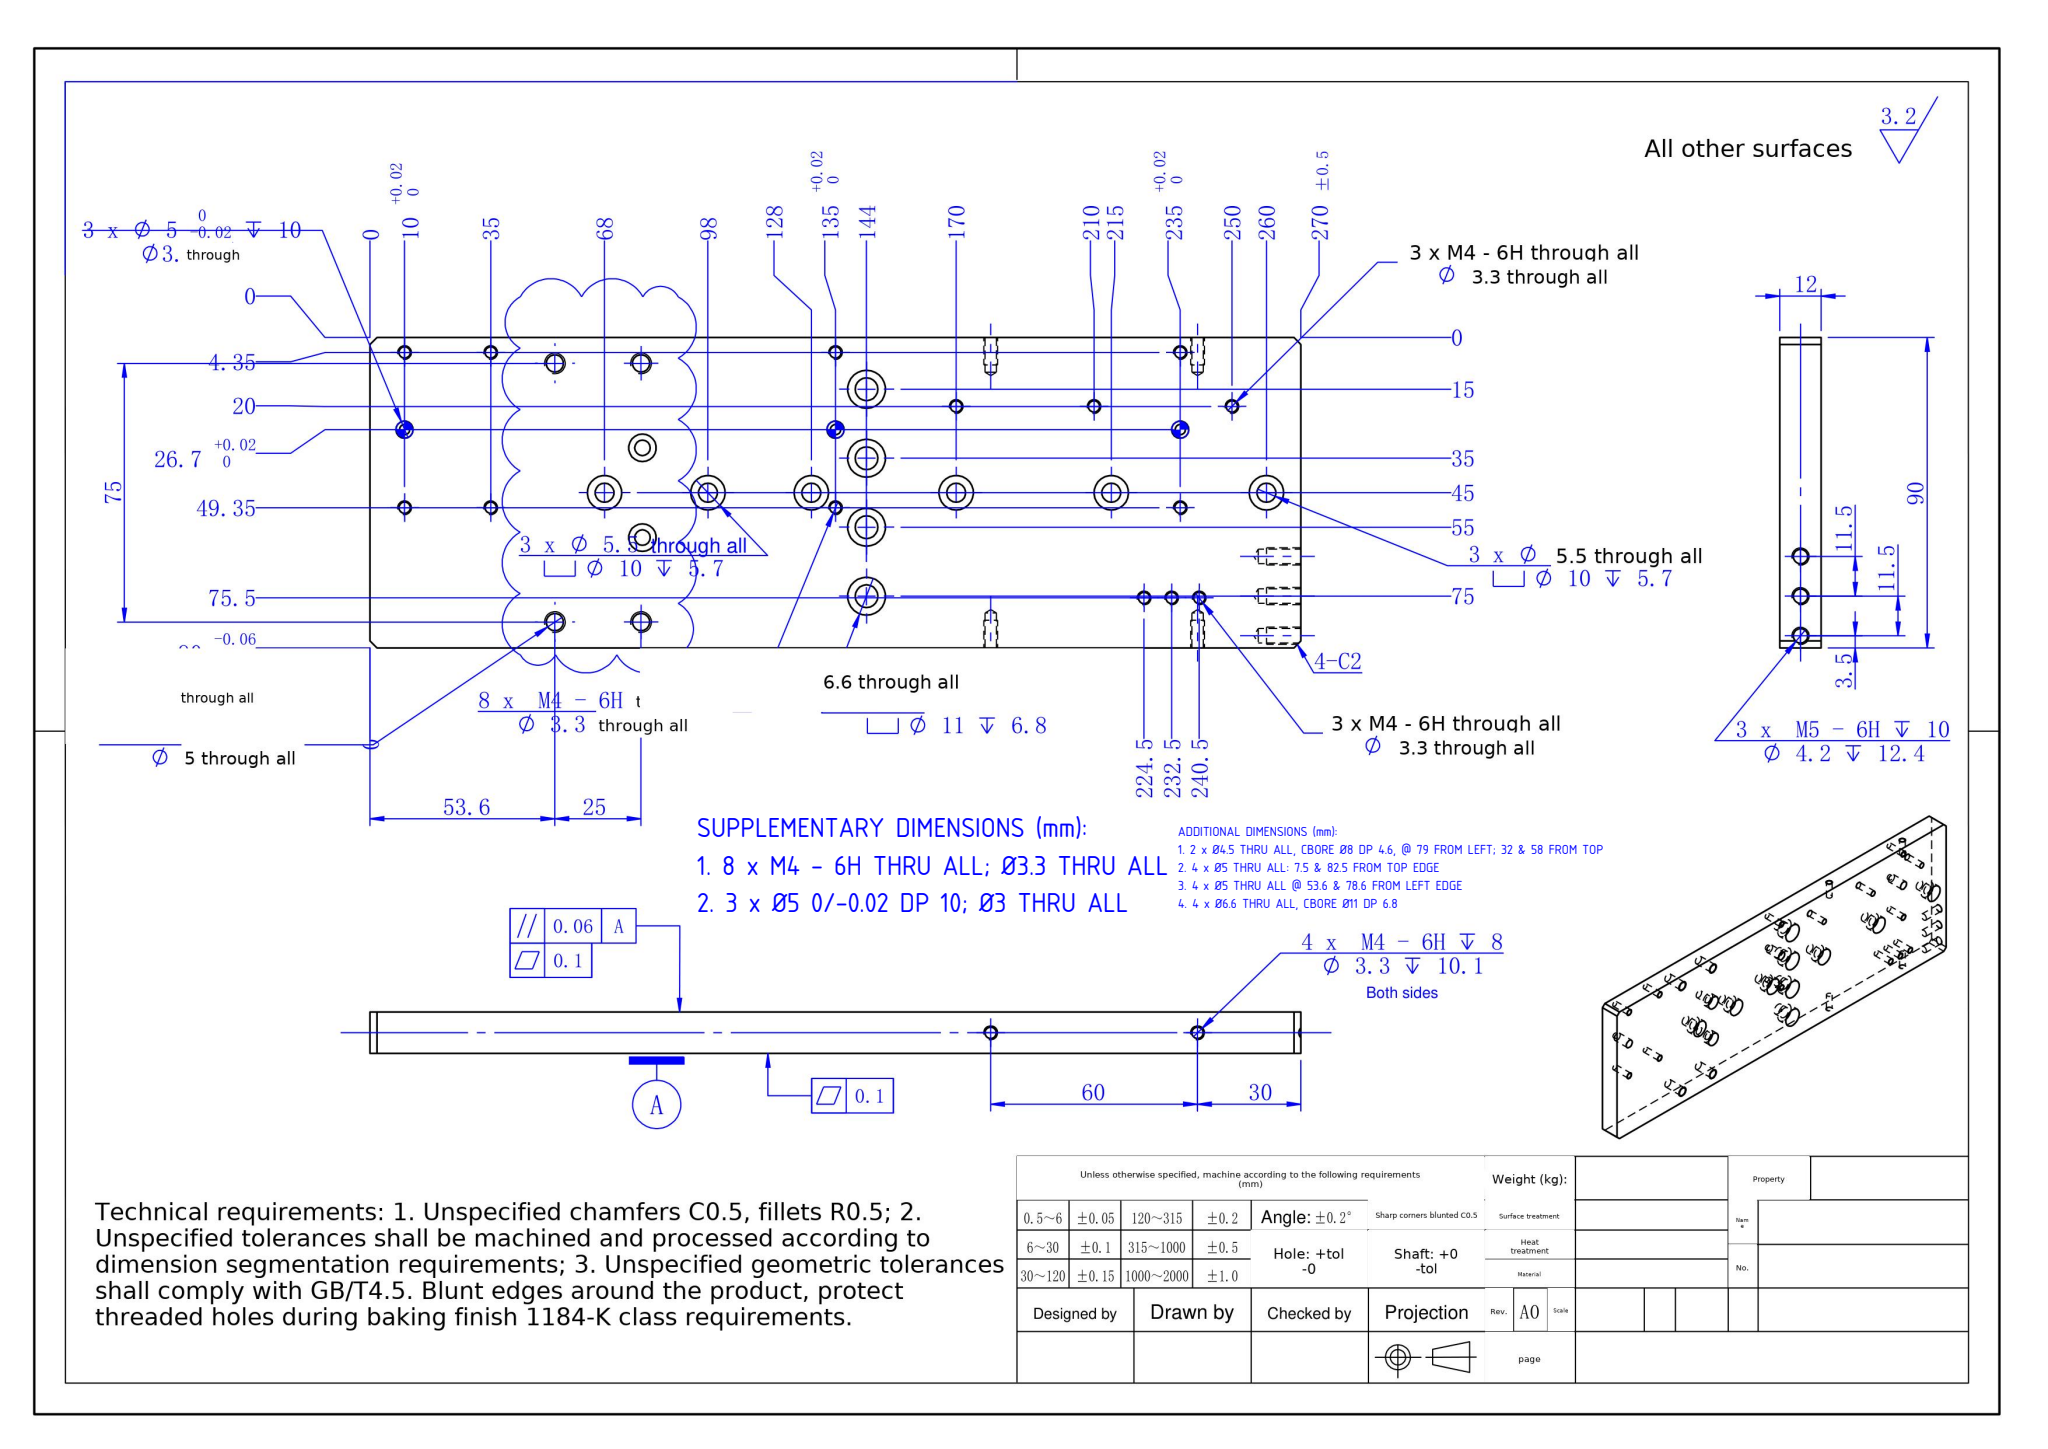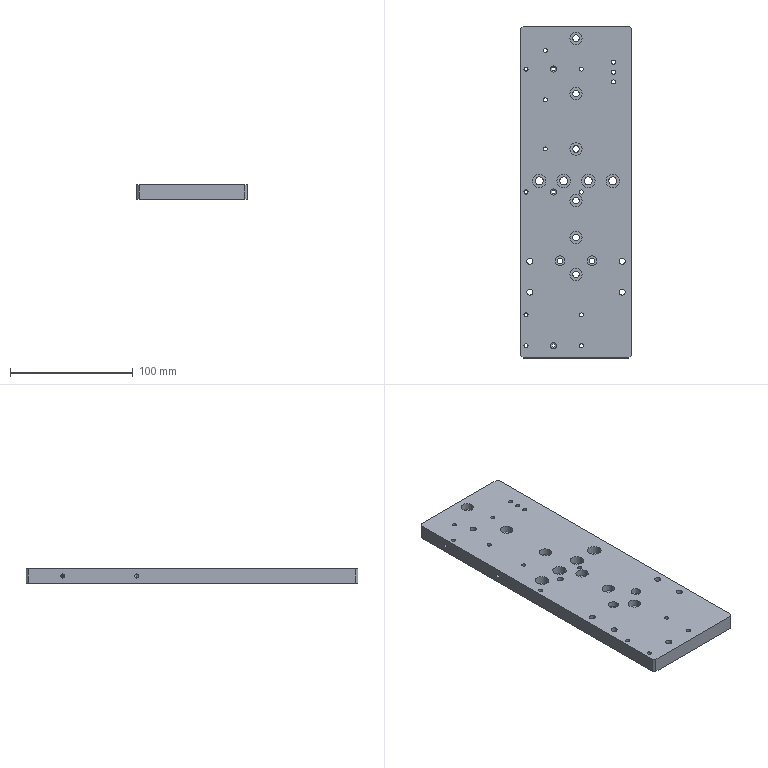Part | SolidWorks | mm | 1 solid | 152 faces | box 90 x 270 x 12 mm | volume 280015 mm3 | cylinder 110 | plane 22 | cone 20 | commonest cylinder face diameters 3.3 x36 5 x14 10 x12 5.5 x12 11 x8 6.6 x8 3 x6 4.2 x6
build123d program:
from build123d import *

# Parameters (mm, degrees)
SKETCH1_W                                         = 90
SKETCH1_H                                         = 270
BOSS_EXTRUDE1_DEPTH                               = 6
CHAMFER1_SIZE                                     = 2
M4_TAPPED_HOLE1_D                                 = 3.3
M4_TAPPED_HOLE2_AT_2_COUNT                        = 2
M4_TAPPED_HOLE2_AT_2_PITCH                        = 60
M5_TAPPED_HOLE1_D                                 = 4.2
M5_TAPPED_HOLE1_DEPTH                             = 12.4
M5_TAPPED_HOLE1_TIP                               = 1.262
M4_TAPPED_HOLE3_D                                 = 3.3
HOLE_SIZE_ACCORDING_TO_HEXAGON_SOCKET_D           = 6.6
HOLE_SIZE_ACCORDING_TO_HEXAGON_SOCKET_CBORE_D     = 11
HOLE_SIZE_ACCORDING_TO_HEXAGON_SOCKET_CBORE_DEPTH = 6.8
HOLE_SIZE_ACCORDING_TO_HEXAGON_SO_2_D             = 5.5
HOLE_SIZE_ACCORDING_TO_HEXAGON_SO_2_CBORE_D       = 10
HOLE_SIZE_ACCORDING_TO_HEXAGON_SO_2_CBORE_DEPTH   = 5.7
HOLE_SIZE_ACCORDING_TO_HEXAGON_SO_3_D             = 5.5
HOLE_SIZE_ACCORDING_TO_HEXAGON_SO_3_CBORE_D       = 10
HOLE_SIZE_ACCORDING_TO_HEXAGON_SO_3_CBORE_DEPTH   = 5.7
M4_TAPPED_HOLE4_D                                 = 3.3
F_3_0_3_DIAMETER_HOLE1_D                          = 3
SIZE_MM_DOWEL_PIN_HOLE_2_D                        = 5
SIZE_MM_DOWEL_PIN_HOLE_2_DEPTH                    = 10
SIZE_MM_DOWEL_PIN_HOLE_2_TIP                      = 1.502
HOLE_SIZE_ACCORDING_TO_HEXAGON_SO_4_D             = 4.5
HOLE_SIZE_ACCORDING_TO_HEXAGON_SO_4_CBORE_D       = 8
HOLE_SIZE_ACCORDING_TO_HEXAGON_SO_4_CBORE_DEPTH   = 4.6
M6_TAPPED_HOLE1_D                                 = 5


with BuildPart() as part:
    # Sketch1 → Boss-Extrude1 (new, symmetric)
    with BuildSketch(Plane.XY):
        Rectangle(SKETCH1_W, SKETCH1_H)
    extrude(amount=BOSS_EXTRUDE1_DEPTH, both=True)

    # Chamfer1
    chamfer1_edges = [part.edges().sort_by_distance(p)[0] for p in [
        (45, -135, 0),
        (-45, -135, 0),
        (-45, 135, 0),
        (45, 135, 0),
    ]]
    chamfer(chamfer1_edges, length=CHAMFER1_SIZE)

    # M4 Tapped Hole1 (through all)
    with Locations(Plane.XY.offset(6)):
        with Locations((30.5, 97.5), (30.5, 89.5), (30.5, 105.5)):
            Hole(M4_TAPPED_HOLE1_D / 2)

    # Sketch7 → M4 Tapped Hole2 (revolve, cut)
    with BuildSketch(Plane(origin=(-45, 45, 0), x_dir=(0, 0, 1), z_dir=(0, 1, 0))):
        Polygon((0, 0), (0, 11.091), (1.65, 10.1), (1.65, 0), align=None)
    m4_tapped_hole2 = revolve(axis=Axis((-51.35, 45, 0), (1, 0, 0)), mode=Mode.SUBTRACT)

    # M4 Tapped Hole2 at 2: M4 Tapped Hole2 ×2
    with Locations(*[(0, i * M4_TAPPED_HOLE2_AT_2_PITCH, 0) for i in range(1, M4_TAPPED_HOLE2_AT_2_COUNT)]):
        add(m4_tapped_hole2, mode=Mode.SUBTRACT)

    # M5 Tapped Hole1
    with Locations(Plane(origin=(0, 135, 0), x_dir=(1, 0, 0), z_dir=(0, 1, 0))):
        with Locations((30, 0), (18.5, 0), (41.5, 0)):
            Hole(M5_TAPPED_HOLE1_D / 2, depth=M5_TAPPED_HOLE1_DEPTH)
            with Locations((0, 0, -(M5_TAPPED_HOLE1_DEPTH + M5_TAPPED_HOLE1_TIP / 2))):  # 118° drill point
                Cone(0, M5_TAPPED_HOLE1_D / 2, M5_TAPPED_HOLE1_TIP, mode=Mode.SUBTRACT)

    # Mirror1: M4 Tapped Hole2 across plane
    add(m4_tapped_hole2.mirror(Plane(origin=(0, 0, 0), x_dir=(0, 0, 1), z_dir=(1, 0, 0))), mode=Mode.SUBTRACT)

    # Mirror1 copy 1 sketch → Mirror1 copy 1 (revolve, cut)
    with BuildSketch(Plane(origin=(45, 105, 0), x_dir=(0, 0, 1), z_dir=(0, 1, 0))):
        Polygon((0, 0), (0, -11.091), (1.65, -10.1), (1.65, 0), align=None)
    revolve(axis=Axis((51.35, 105, 0), (1, 0, 0)), mode=Mode.SUBTRACT)

    # M4 Tapped Hole3 (through all)
    with Locations(Plane(origin=(0, 0, -6), x_dir=(-1, 0, 0), z_dir=(0, 0, -1))):
        with Locations((25, 115), (25, 75), (25, 35)):
            Hole(M4_TAPPED_HOLE3_D / 2)

    # Hole Size _ According to_ Hexagon Socket (through all)
    with Locations(Plane.XY.offset(6)):
        with Locations((30, 9), (10, 9), (-10, 9), (-30, 9)):
            CounterBoreHole(HOLE_SIZE_ACCORDING_TO_HEXAGON_SOCKET_D / 2, HOLE_SIZE_ACCORDING_TO_HEXAGON_SOCKET_CBORE_D / 2, HOLE_SIZE_ACCORDING_TO_HEXAGON_SOCKET_CBORE_DEPTH)

    # Hole Size _ According to_ Hexagon So 2 (through all)
    with Locations(Plane.XY.offset(6)):
        with Locations((0, 35), (0, 80), (0, 125)):
            CounterBoreHole(HOLE_SIZE_ACCORDING_TO_HEXAGON_SO_2_D / 2, HOLE_SIZE_ACCORDING_TO_HEXAGON_SO_2_CBORE_D / 2, HOLE_SIZE_ACCORDING_TO_HEXAGON_SO_2_CBORE_DEPTH)

    # Hole Size _ According to_ Hexagon So 3 (through all)
    with Locations(Plane.XY.offset(6)):
        with Locations((0, -7), (0, -37), (0, -67)):
            CounterBoreHole(HOLE_SIZE_ACCORDING_TO_HEXAGON_SO_3_D / 2, HOLE_SIZE_ACCORDING_TO_HEXAGON_SO_3_CBORE_D / 2, HOLE_SIZE_ACCORDING_TO_HEXAGON_SO_3_CBORE_DEPTH)

    # M4 Tapped Hole4 (through all)
    with Locations(Plane.XY.offset(6)):
        with Locations((-40.65, -125), (-40.65, -100), (4.35, -125), (4.35, -100), (-40.65, 100), (4.35, 100), (4.35, 0), (-40.65, 0)):
            Hole(M4_TAPPED_HOLE4_D / 2)

    # 3.0 _3_ Diameter Hole1 (through all)
    with Locations(Plane(origin=(0, 0, -6), x_dir=(-1, 0, 0), z_dir=(0, 0, -1))):
        with Locations((18.3, 100), (18.3, 0), (18.3, -125)):
            Hole(F_3_0_3_DIAMETER_HOLE1_D / 2)

    # Size mm Dowel Pin Hole 2
    with Locations(Plane.XY.offset(6)):
        with Locations((-18.3, 100), (-18.3, 0), (-18.3, -125)):
            Hole(SIZE_MM_DOWEL_PIN_HOLE_2_D / 2, depth=SIZE_MM_DOWEL_PIN_HOLE_2_DEPTH)
            with Locations((0, 0, -(SIZE_MM_DOWEL_PIN_HOLE_2_DEPTH + SIZE_MM_DOWEL_PIN_HOLE_2_TIP / 2))):  # 118° drill point
                Cone(0, SIZE_MM_DOWEL_PIN_HOLE_2_D / 2, SIZE_MM_DOWEL_PIN_HOLE_2_TIP, mode=Mode.SUBTRACT)

    # Hole Size _ According to_ Hexagon So 4 (through all)
    with Locations(Plane.XY.offset(6)):
        with Locations((13, -56), (-13, -56)):
            CounterBoreHole(HOLE_SIZE_ACCORDING_TO_HEXAGON_SO_4_D / 2, HOLE_SIZE_ACCORDING_TO_HEXAGON_SO_4_CBORE_D / 2, HOLE_SIZE_ACCORDING_TO_HEXAGON_SO_4_CBORE_DEPTH)

    # M6 Tapped Hole1 (through all)
    with Locations(Plane.XY.offset(6)):
        with Locations((-37.5, -81.4), (37.5, -81.4), (-37.5, -56.4), (37.5, -56.4)):
            Hole(M6_TAPPED_HOLE1_D / 2)


solid = part.part